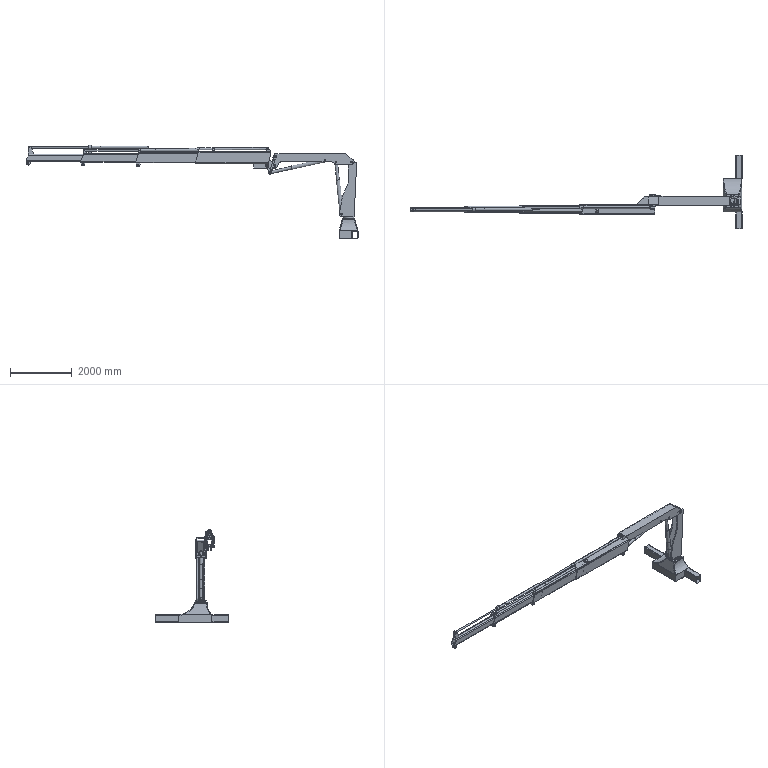Assembly | NX | mm | 37 component files | 41 solids | 919 faces | box 10753.2 x 2378 x 3016.7 mm | volume 477244886 mm3 | plane 425 | cylinder 320 | other 124 | cone 24 | spline 22 | torus 4 | commonest cylinder face diameters 279.4 x60 50.8 x46 25.4 x42 50 x30 101.6 x14 76.2 x13 30 x10 20 x10
Bill of materials:
unnamed part 1 | 1 |  | Solid straight cylindrical pin with chamfered edges at both ends; slender (length roughly 6x diameter).
unnamed part 2 | 2 |  | Short solid round rod with a flat, thinner tab at one end; the tab has a rounded end and a through hole (eye end).
unnamed part 3 | 1 |  | Long, slender solid round rod with a flat eye tab at one end (rounded tab with a small through hole); other end plain and flat.
unnamed part 4 | 2 |  | Long, slender solid round rod with a flat eye tab at one end (rounded tab with small through hole); other end plain.
unnamed part 5 | 1 |  | Solid cylindrical pin with chamfered ends; somewhat stockier than unnamed part 1.
unnamed part 6 | 2 |  | Solid cylindrical pin with chamfered ends; slightly larger diameter-to-length ratio than the other pins.
unnamed part 7 | 1 |  | Long formed channel (inverted U section) arm with a profiled side outline; side walls extend past the web at both ends as paired lugs, with several through holes in the side walls.
unnamed part 8 | 2 |  | Thick annular ring (spacer/washer-like) with a central through bore; plain cylindrical outer and inner surfaces.
unnamed part 9 | 1 |  | Square flange plate with rounded corners, four corner through holes, and a central raised circular boss with a large through bore; the boss periphery carries a ring of small teeth/serrations and a fillet at its base.
unnamed part 10 | 1 |  | Hollow rectangular tube with rounded corners and angled-cut ends; at one end two parallel upright plate lugs with holes project above, and two lugs with holes project below.
unnamed part 11 | 1 |  | Hollow rectangular tube with rounded corners and angled ends; one end carries a thick lug with a large hole plus two thin parallel plates above, and two thin lugs with a small hole below.
unnamed part 12 | 1 |  | Long slender round rod with a flat eye tab (small through hole) at one end and a thin longitudinal raised rib or line running along most of its length.
unnamed part 13 | 1 |  | Tall bracket made from two parallel plates. The plates share a side profile that tapers and curves, with a rounded lug at the top and another at the bottom corner. The pair sits on a round disc or collar with a large central bore.
unnamed part 14 | 1 |  | Long hollow tube of rectangular section with rounded corners and angled cut ends. A slotted ring (C-shaped sleeve) sits on the top face near one end, and two parallel holed lugs project upward at the other end.
unnamed part 15 | 1 |  | Short solid cylindrical pin with chamfers at both ends, roughly three times as long as its diameter.
unnamed part 16 | 1 |  | Rectangular hollow tube with a raised boss. The boss flares up from the tube through concave curved transitions and ends in a square flange plate with a large central bore and four small corner holes.
unnamed part 17 | 1 |  | Wedge-shaped bracket block with a sloped top face. It ends in a fork of two parallel lugs with rounded tips, and each lug has holes.
unnamed part 18 | 2 |  | Long, slender, straight cylindrical rod with plain ends.
unnamed part 19 | 4 |  | Solid cylindrical pin with chamfers at both ends, roughly four times as long as its diameter.
unnamed part 20 | 2 |  | Slender solid cylindrical pin with small chamfers at both ends, roughly six to seven times as long as its diameter.
unnamed part 21 | 1 |  | Long hollow tube of rectangular section with rounded corners and angled ends. Near one end it carries attachments on both faces: on one face, a holed tab and a ring boss on a stem; on the opposite face, two parallel holed lugs.
unnamed part 22 | 2 |  | Long solid cylindrical rod with a small ring or eye at one end.
unnamed part 23 | 2 |  | Flat link plate of constant thickness. It has two rounded ends, each with a large through-hole, joined by a narrower angled web, giving an offset dog-bone outline.
unnamed part 24 | 2 |  | Thin, flat, elongated link plate with rounded ends, each with a through-hole, joined by a long narrow web. The outline is slightly offset (S-like).
unnamed part 25 | 1 |  | Solid straight cylindrical rod with a small chamfer on both ends; it is about 5 times as long as it is wide. Its shape matches a plain pin, but no assembly role is confirmed.
Mates:
1. touch align | support_arm 1 face | base_pad 1 face
2. touch align | support_arm 1 face | base_pad 1 face
3. touch align | ext_arm 1 face | support_arm 1 face
4. touch align | ext_arm 1 face | support_arm 1 face
5. touch align | connector 1 face | ext_arm 1 face
6. touch align | connector 1 face | ext_arm 1 face
7. touch align | arm_section_1 1 face | connector 1 face
8. touch align | arm_section_2 1 face | arm_section_1 1 face
9. touch align | arm_section_2 1 face | arm_section_1 1 face
10. touch align | arm_section_3 1 face | arm_section_2 1 face
11. touch align | arm_section_3 1 face | arm_section_2 1 face
12. touch align | arm_section_4 1 face | arm_section_3 1 face
13. touch align | arm_section_4 1 face | arm_section_3 1 face
14. touch align | pin_304 4 face | connector 1 face
15. touch align | pin_304 4 face | ext_arm 1 face
16. touch align | pin_304 3 face | ext_arm 1 face
17. touch align | pin_304 2 face | ext_arm 1 face
18. touch align | pin_304 1 face | support_arm 1 face
19. touch align | pin_330 1 face | ext_arm 1 face
20. touch align | pin_254 1 face | support_arm 1 face
21. touch align | pin_254 1 face | support_arm 1 face
22. touch align | pin_127 2 face | arm_section_1 1 face
23. touch align | pin_127 2 face | arm_section_1 1 face
24. touch align | pin_76 1 face | arm_section_2 1 face
25. touch align | pin_76 1 face | arm_section_2 1 face
26. touch align | pin_152 1 face | arm_section_3 1 face
27. touch align | pin_152 1 face | arm_section_3 1 face
28. touch align | pin_127 1 face | arm_section_4 1 face
29. touch align | large_arm_ext_rod 2 face | pin_304 2 face
30. touch align | large_arm_cyl_body 2 face | pin_254 1 face
31. touch align | washer 1 face | connector 1 face
32. touch align | connector_1 2 face | washer 2 face
33. touch align | connector_1 1 face | washer 1 face
34. touch align | pin_381 2 face | connector_1 1 face
35. touch align | pin_381 1 face | connector_1 1 face
36. touch align | connector_2 2 face | connector_1 2 face
37. touch align | connector_2 1 face | connector_1 1 face
38. touch align | cyl_body 1 face | pin_127 2 face
39. touch align | mid_arm_ext_rod 1 face | cyl_body 1 face
40. touch align | mid_arm_ext_rod 1 face | arm_section_2 1 face
41. touch align | small_arm_ext_rod 2 face | pin_152 1 face
42. touch align | small_arm_ext_rod 2 face | arm_section_3 1 face
43. touch align | cyl_body_2 2 face | small_arm_ext_rod 2 face
44. touch align | small_arm_ext_rod 1 face | pin_127 1 face
45. touch align | cyl_body_2 1 face | small_arm_ext_rod 1 face
46. touch align | large_arm_ext_rod 1 face | large_arm_cyl_body 1 face
47. touch align | large_arm_cyl_body 1 face | pin_304 3 face
48. fix | ext_arm 1 component
49. touch align | large_arm_ext_rod 1 face | pin_381 1 face